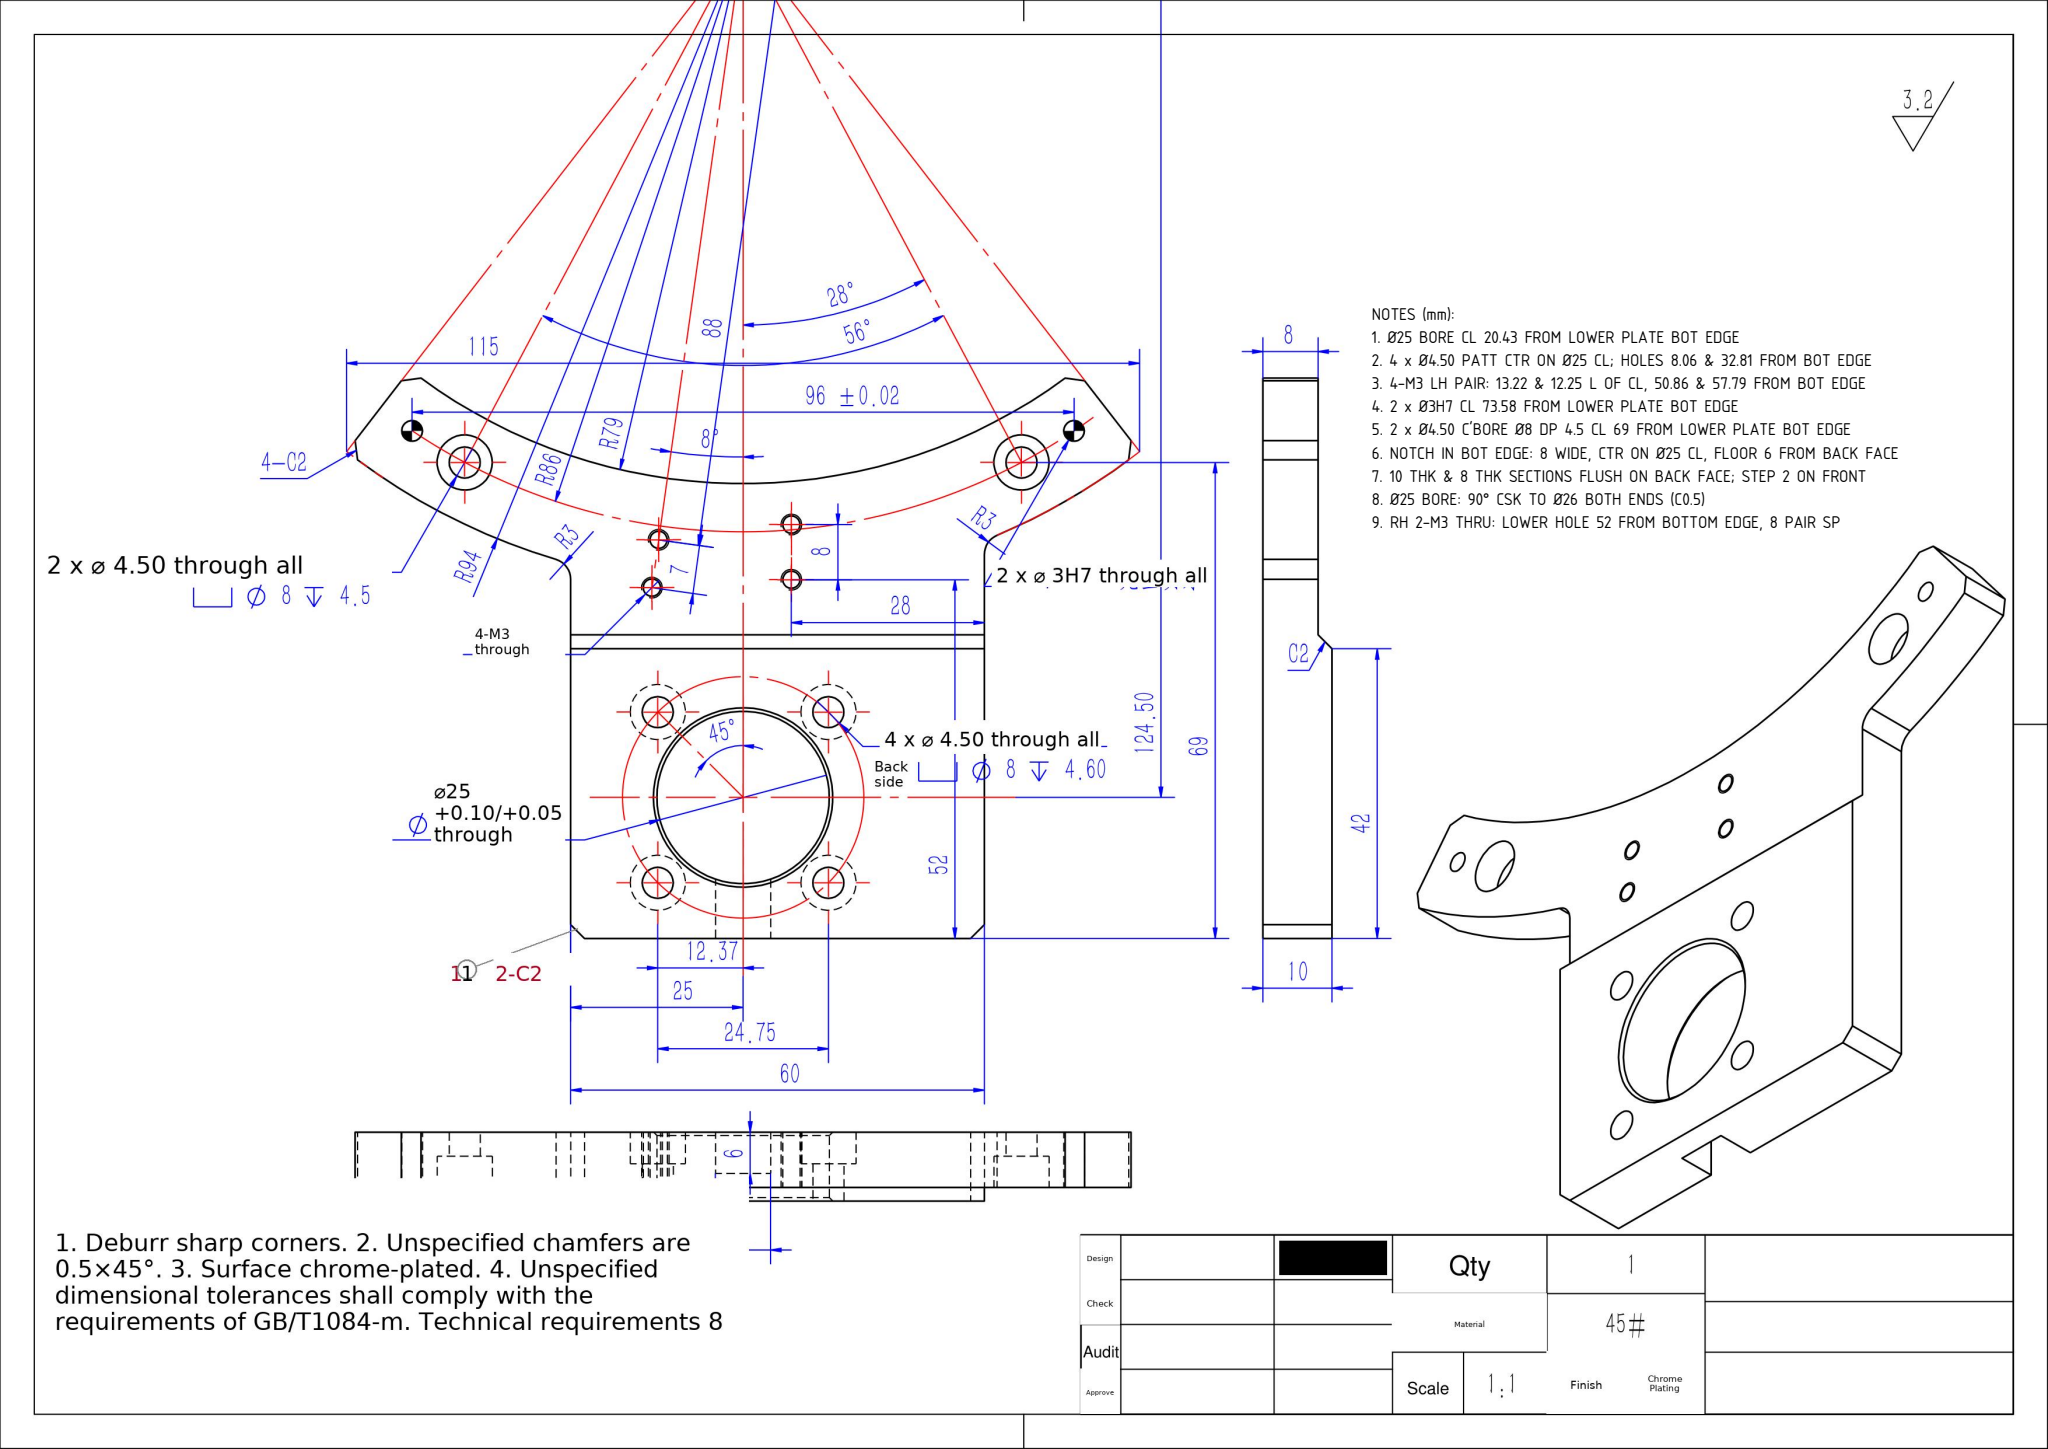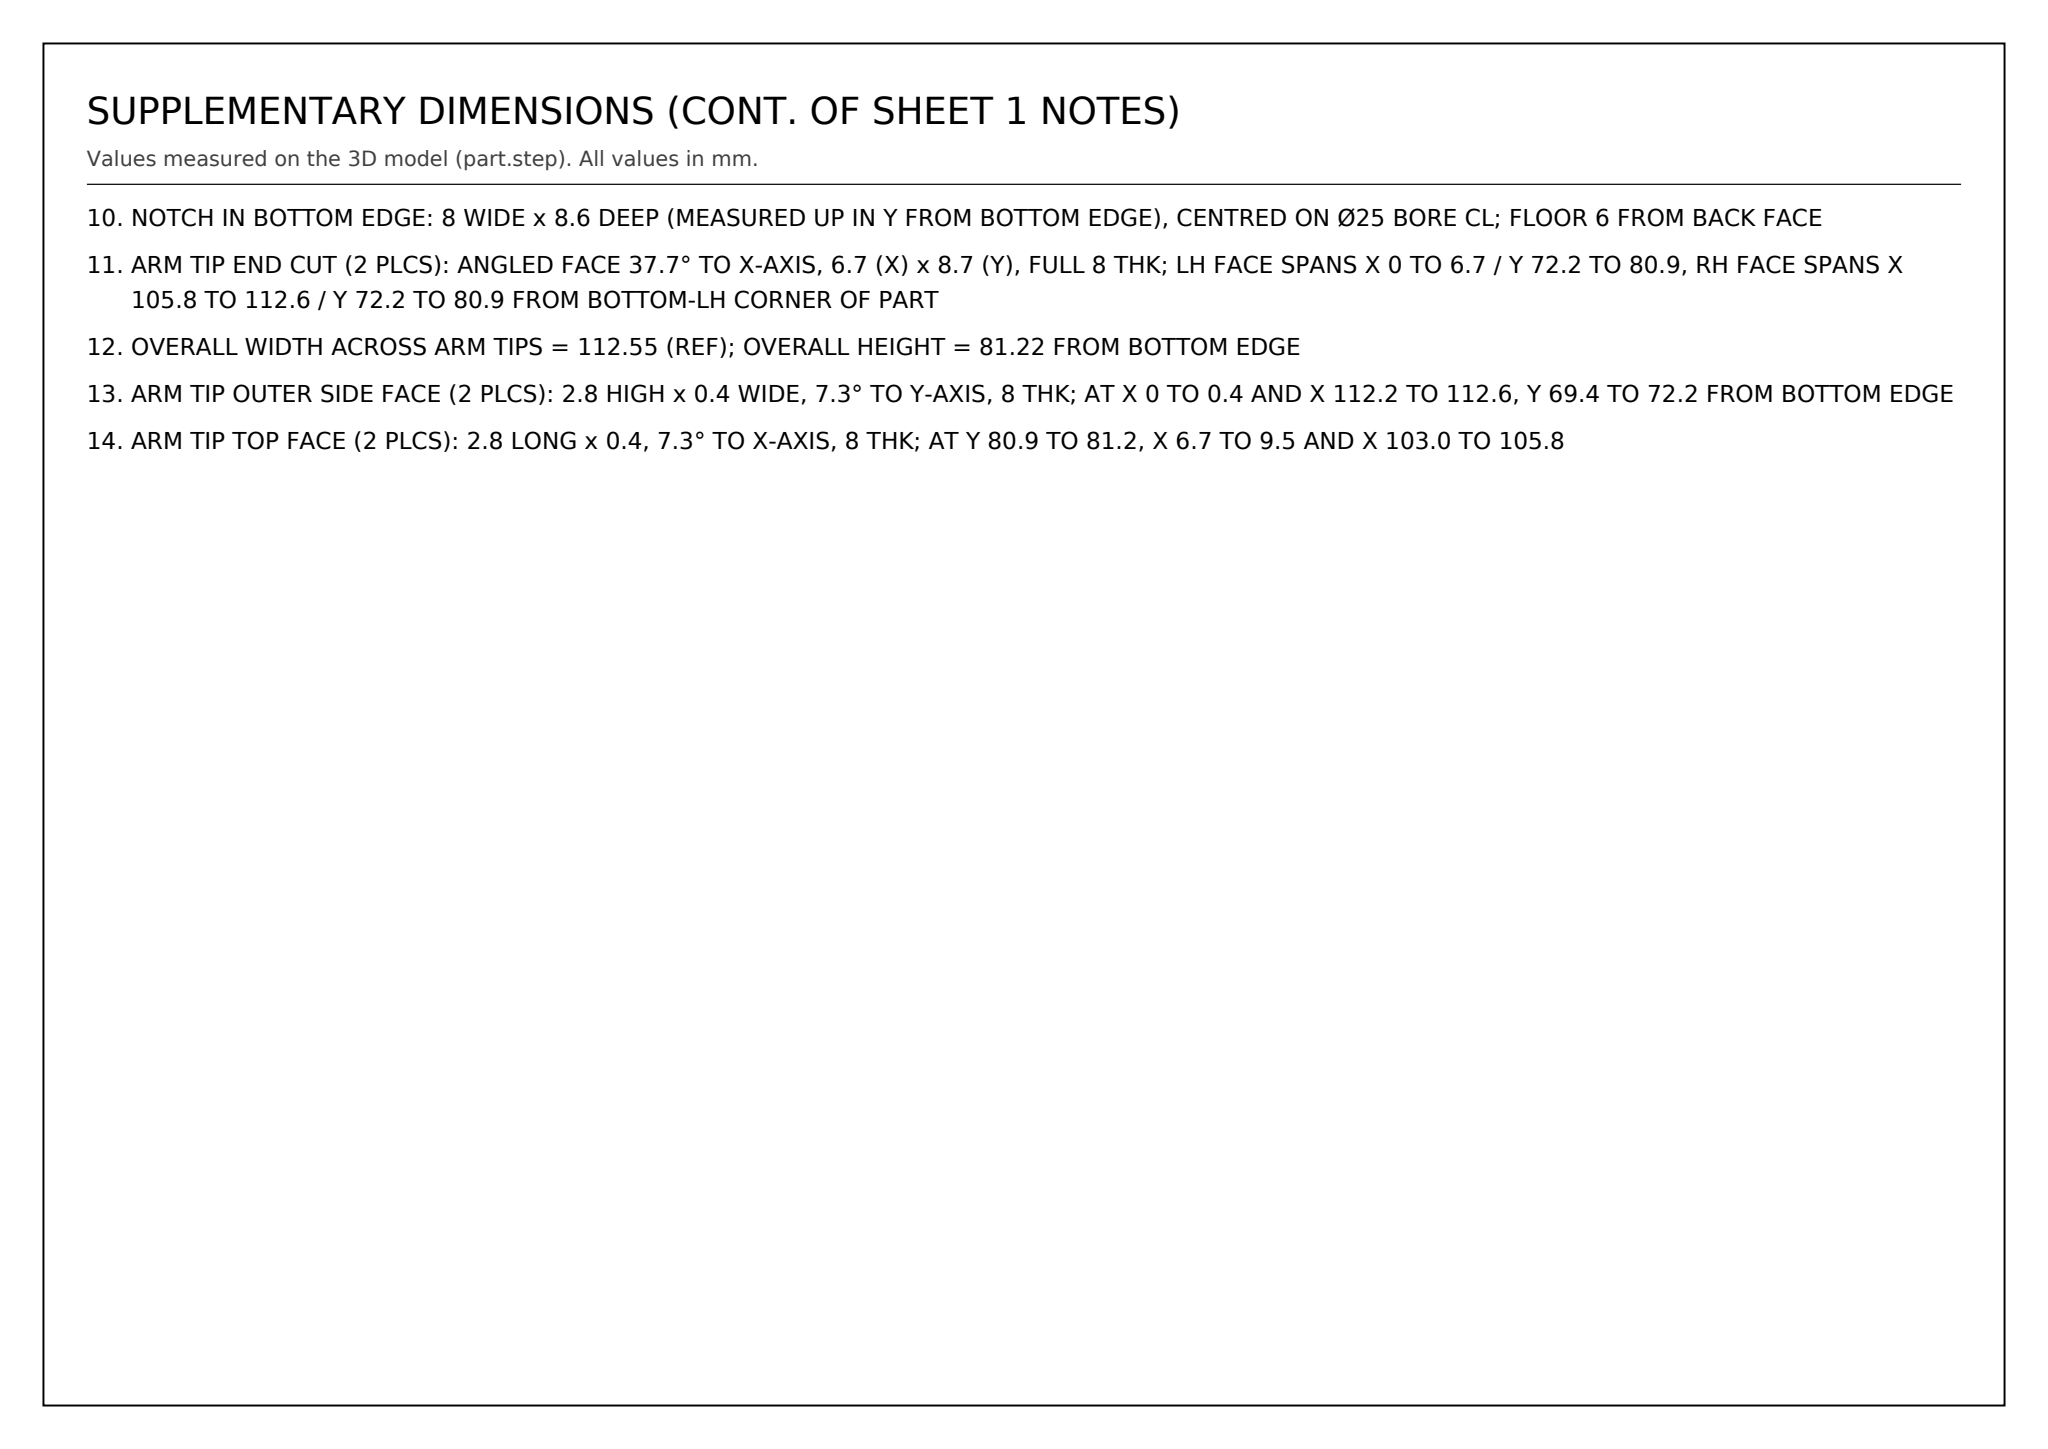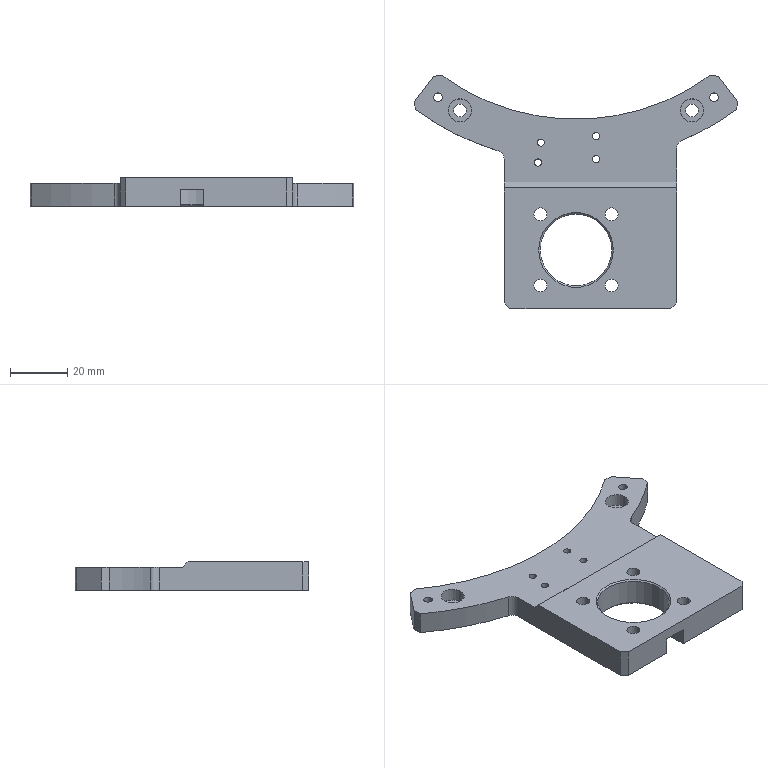Part | SolidWorks | mm | 1 solid | 72 faces | box 112.55 x 81.22 x 10 mm | volume 36606 mm3 | cylinder 43 | plane 24 | cone 5 | commonest cylinder face diameters 8 x12 4.5 x12 2.5 x8 3 x4 25 x2 188 x2 6 x2 158 x1
Drawing notes:
Ø25 BORE CL 20.43 FROM LOWER PLATE BOT EDGE | from the solid: Ø25 cyl axis at y=20.43, bbox min y=0 = plate bottom edge
4 x Ø4.50 PATT CTR ON Ø25 CL; HOLES 8.06 & 32.81 FROM BOT EDGE | from the solid: Ø4.5 c'bored holes at y=8.06 & 32.81 (ctr 20.435 = Ø25 ctr), x=43.9/68.65
4-M3 LH PAIR: 13.22 & 12.25 L OF CL, 50.86 & 57.79 FROM BOT EDGE | from the solid: Ø2.5 holes at (43.06,50.86) & (44.03,57.79); CL x=56.28, bot edge y=0
2 x Ø3H7 CL 73.58 FROM LOWER PLATE BOT EDGE | from the solid: Ø3 holes at (8.28,73.58) & (104.28,73.58), symmetric ±48 about CL x=56.28
2 x Ø4.50 C'BORE Ø8 DP 4.5 CL 69 FROM LOWER PLATE BOT EDGE | from the solid: Ø4.5/Ø8 c'bore at (15.9,69) & (96.65,69); spacing 80.75 about CL
NOTCH IN BOT EDGE: 8 WIDE, CTR ON Ø25 CL, FLOOR 6 FROM BACK FACE | from the solid: x-planes 52.28 & 60.28 (8 wide, ctr 56.28 = CL); z-plane 6.0
10 THK & 8 THK SECTIONS FLUSH ON BACK FACE; STEP 2 ON FRONT | from the solid: z-planes 8.0 (arm face) and 10.0 (plate face), common back face z=0
Ø25 BORE: 90° CSK TO Ø26 BOTH ENDS (C0.5) | from the solid: cones 90° ref Ø26 x2 on Ø25 bore; bore cyl len 9 + 2 x 0.5 = 10 thk
RH 2-M3 THRU: LOWER HOLE 52 FROM BOTTOM EDGE, 8 PAIR SP | from the solid: Ø2.5 z-holes at (63.28,52.0) and (63.28,60.0); bbox min y = bottom edge 0
NOTCH IN BOTTOM EDGE: 8 WIDE x 8.6 DEEP (MEASURED UP IN Y FROM BOTTOM EDGE), CENTRED ON Ø25 BORE CL; FLOOR 6 FROM BACK FACE | from the solid: axis_planes x=52.3 and x=60.3 each extent y[0.0,8.6] z[0.0,6.0] (8 mm apart, notch sides); plane z=6.0 extent x[52.3,60.3] y[0.0,8.6] (notch floor)
ARM TIP END CUT (2 PLCS): ANGLED FACE 37.7° TO X-AXIS, 6.7 (X) x 8.7 (Y), FULL 8 THK; LH FACE SPANS X 0 TO 6.7 / Y 72.2 TO 80.9, RH FACE SPANS X 105.8 TO 112.6 / Y 72.2 TO 80.9 FROM BOTTOM-LH CORNER OF PART | from the solid: inclined_planes: angle_to_xyz_axes [37.7,52.3,90.0], bbox_from [0.0,72.2,0.0] and [105.8,72.2,0.0], size [6.7,8.7,8.0]
OVERALL WIDTH ACROSS ARM TIPS = 112.55 (REF); OVERALL HEIGHT = 81.22 FROM BOTTOM EDGE | from the solid: bbox_xyz [112.553, 81.219, 10.0]
ARM TIP OUTER SIDE FACE (2 PLCS): 2.8 HIGH x 0.4 WIDE, 7.3° TO Y-AXIS, 8 THK; AT X 0 TO 0.4 AND X 112.2 TO 112.6, Y 69.4 TO 72.2 FROM BOTTOM EDGE | from the solid: inclined_planes: angle_to_xyz_axes [7.3,82.7,90.0], bbox_from [0.0,69.4,0.0] and [112.2,69.4,0.0], size [0.4,2.8,8.0]
ARM TIP TOP FACE (2 PLCS): 2.8 LONG x 0.4, 7.3° TO X-AXIS, 8 THK; AT Y 80.9 TO 81.2, X 6.7 TO 9.5 AND X 103.0 TO 105.8 | from the solid: inclined_planes: angle_to_xyz_axes [82.7,7.3,90.0], bbox_from [6.7,80.9,0.0] and [103.0,80.9,0.0], size [2.8,0.4,8.0]